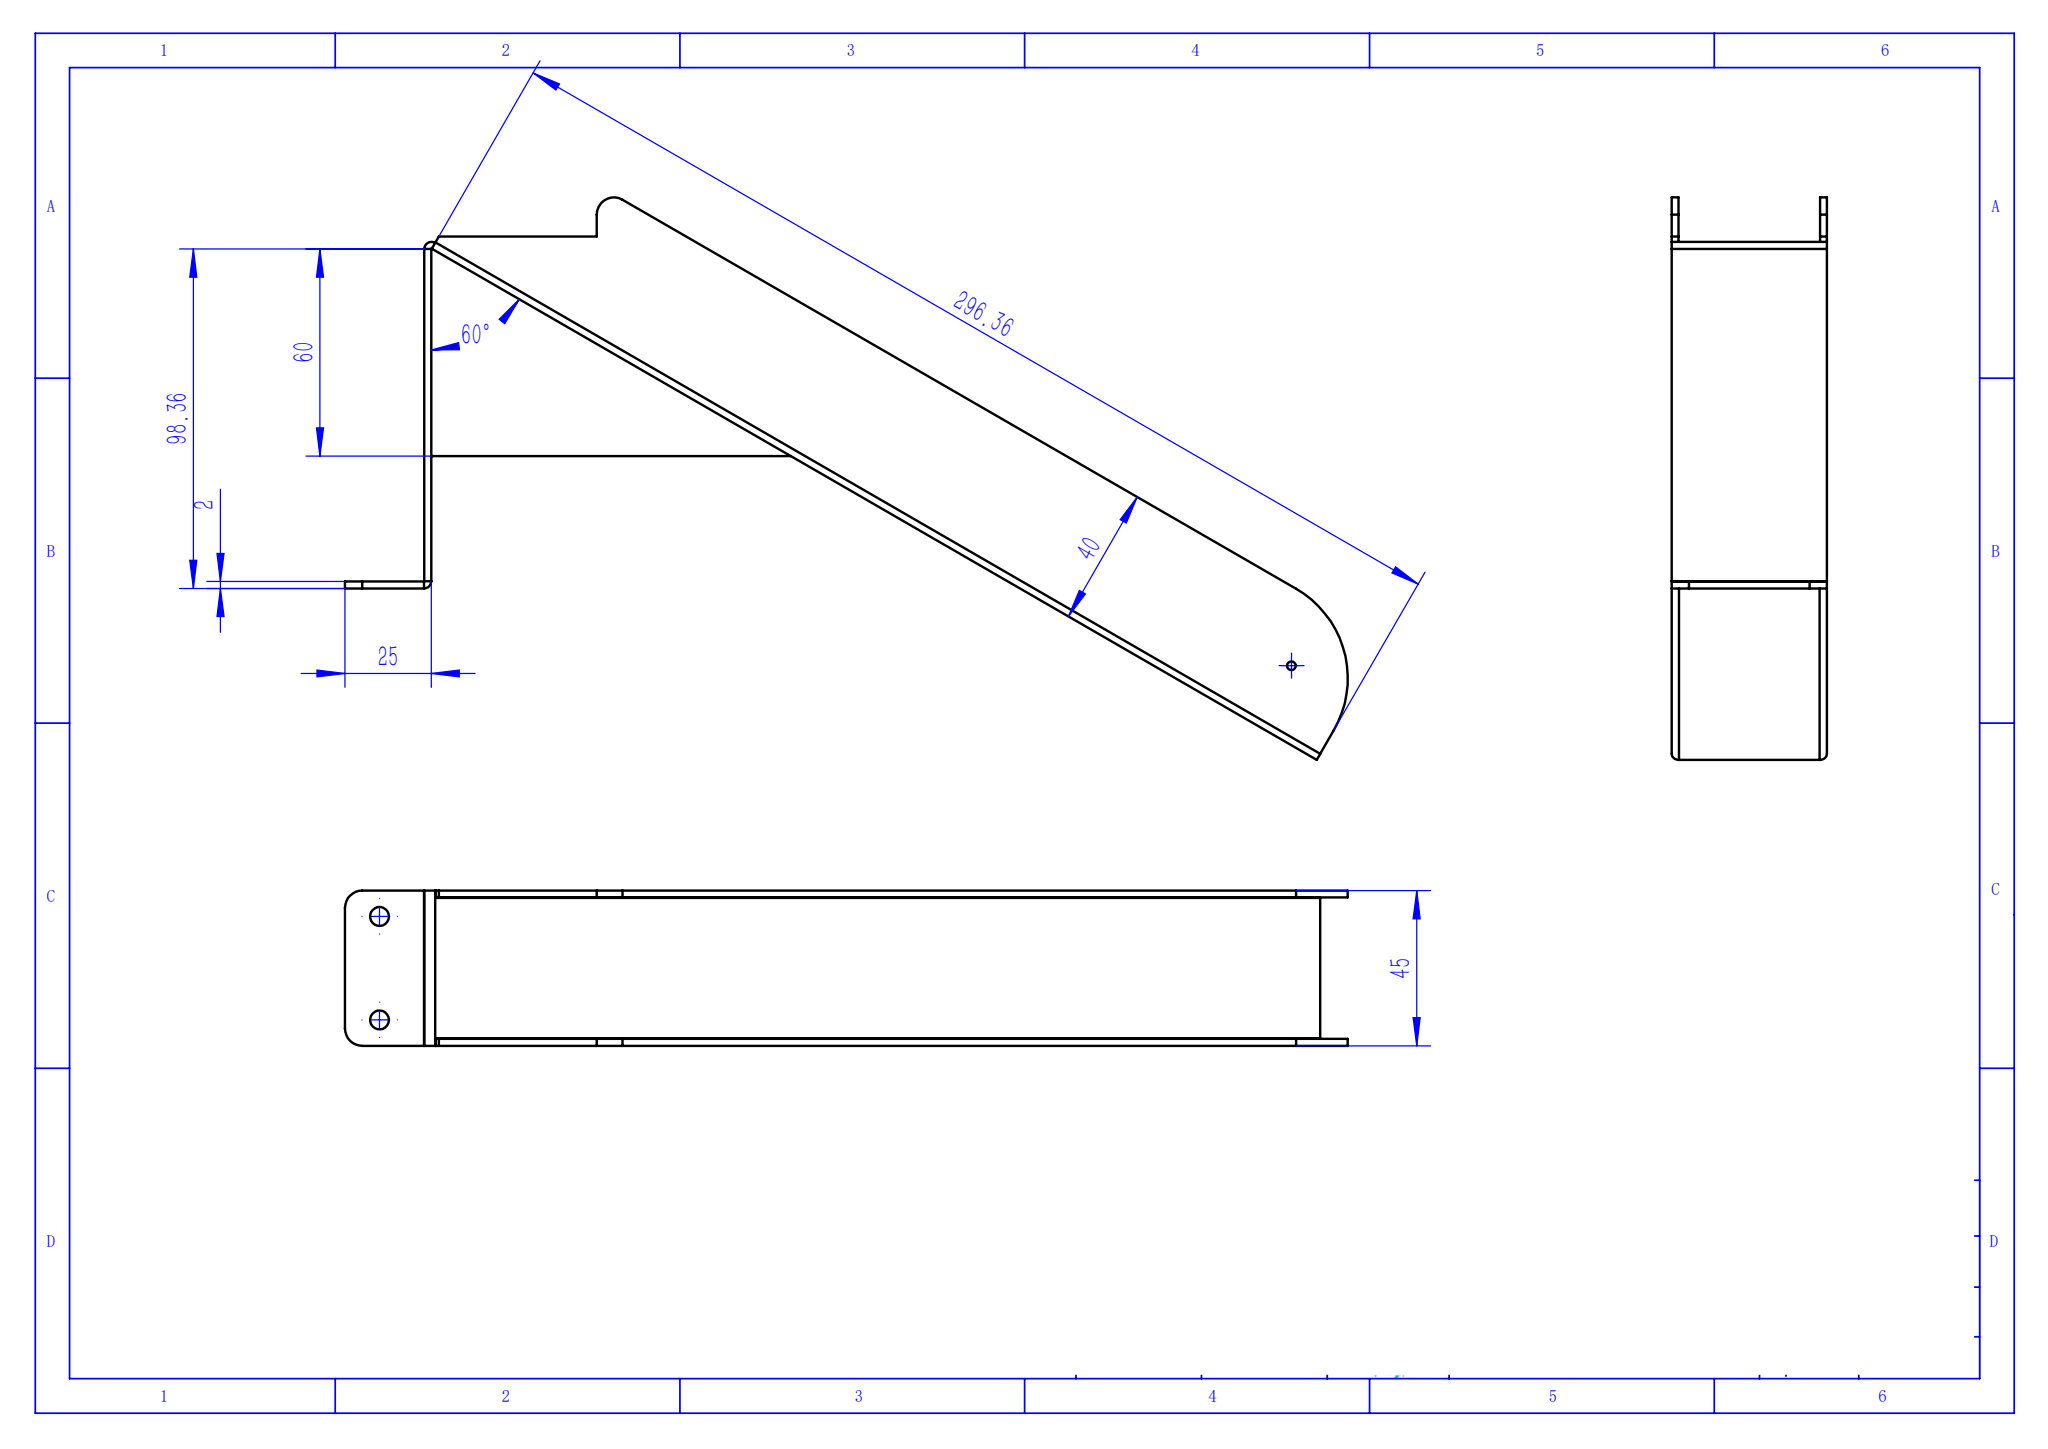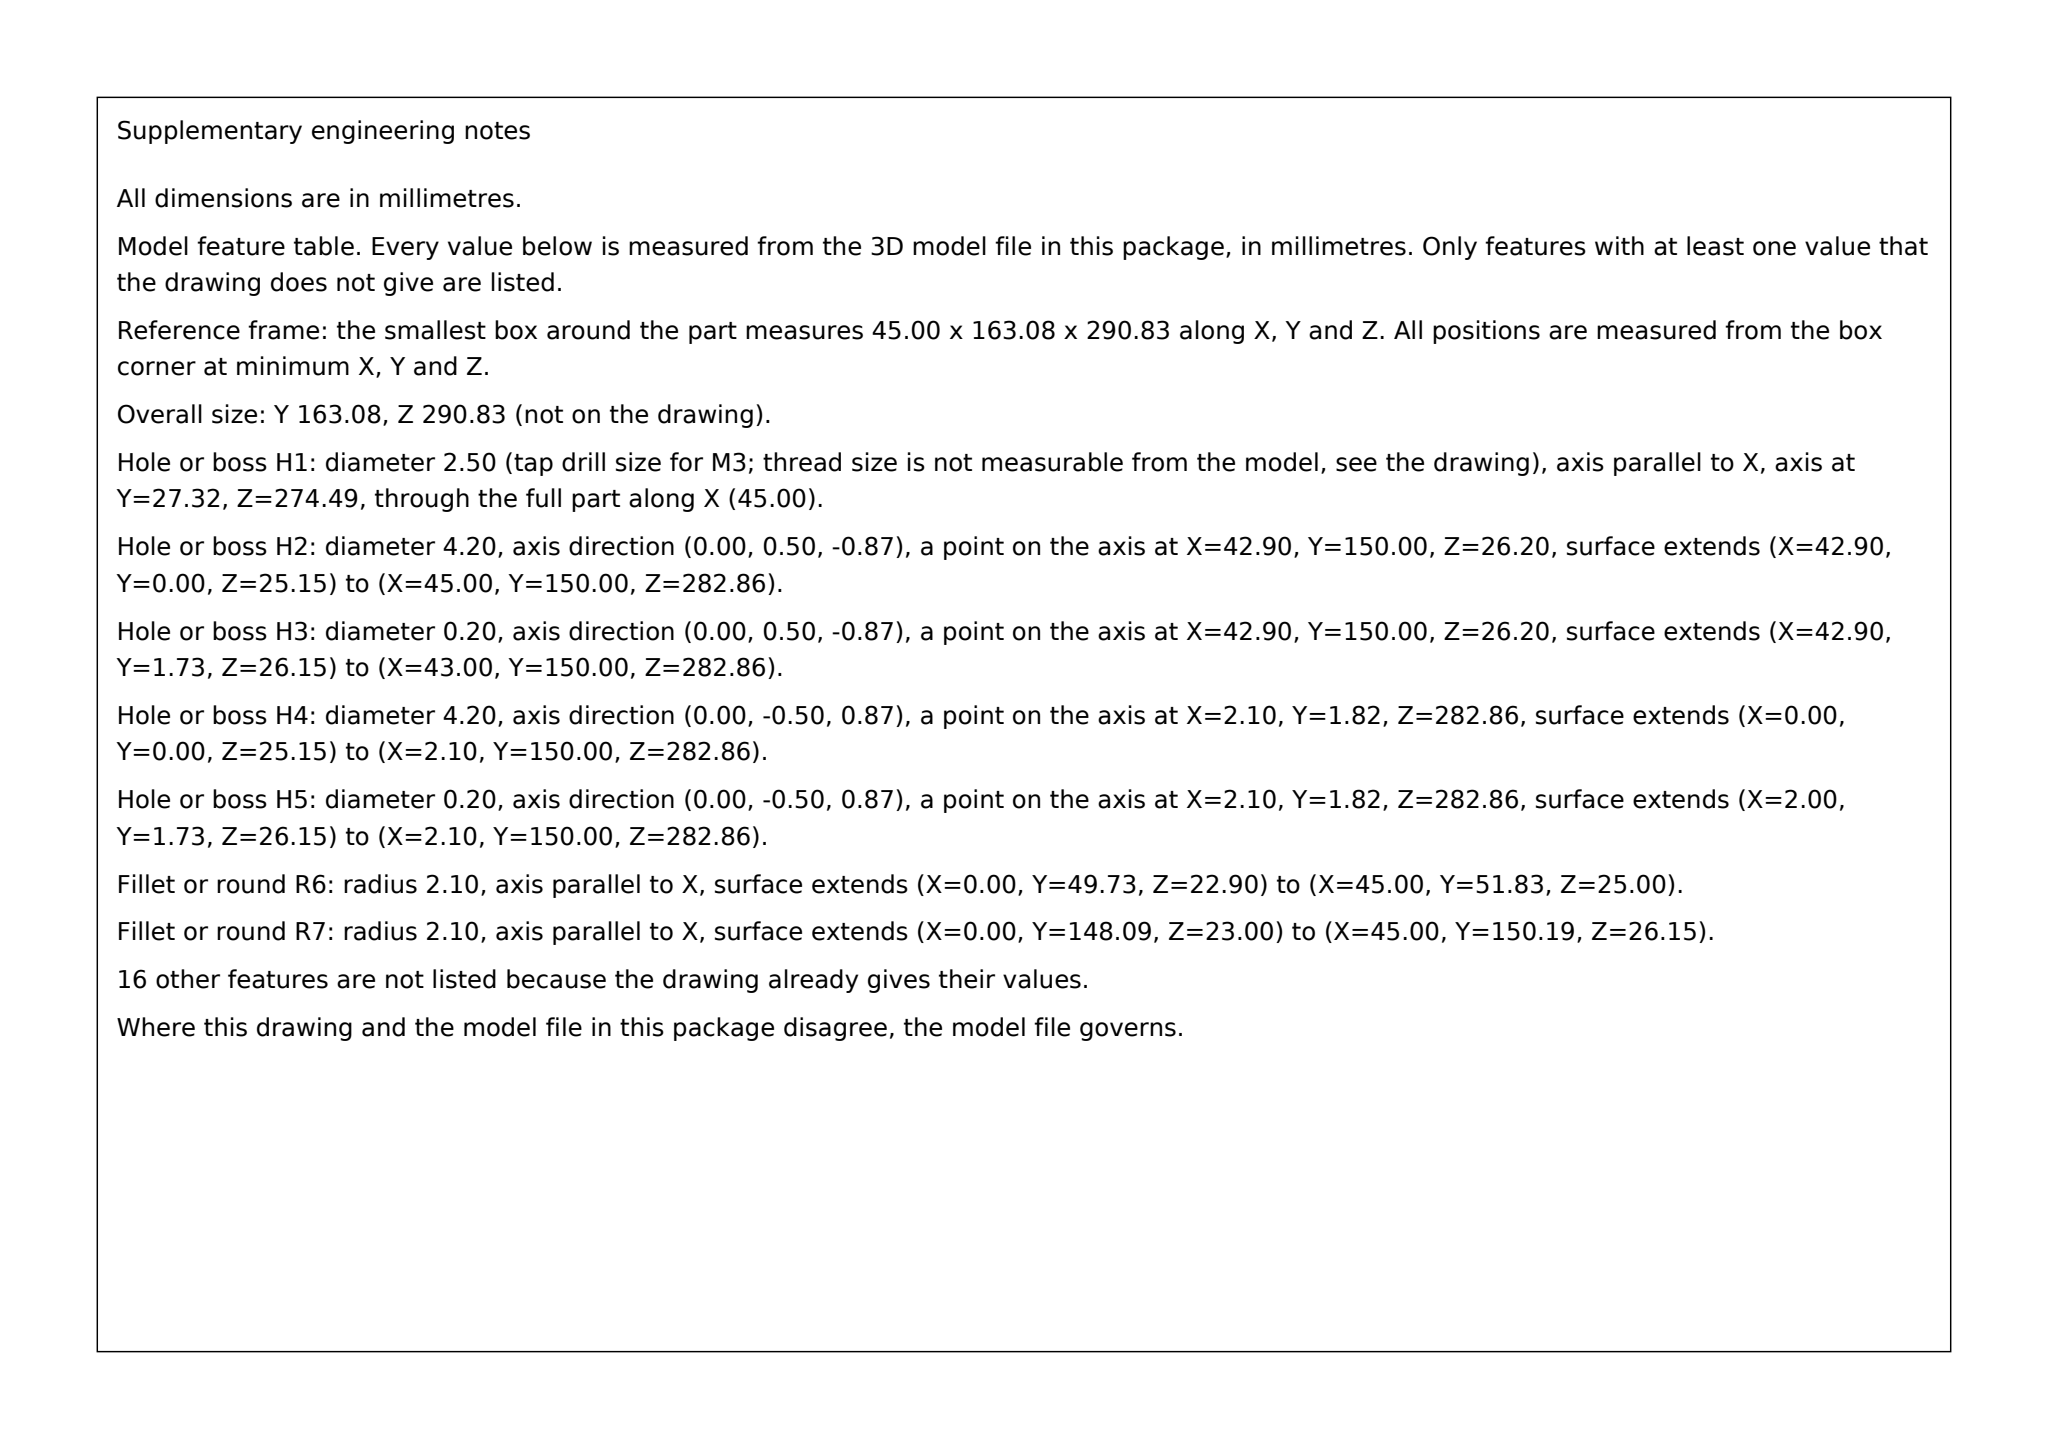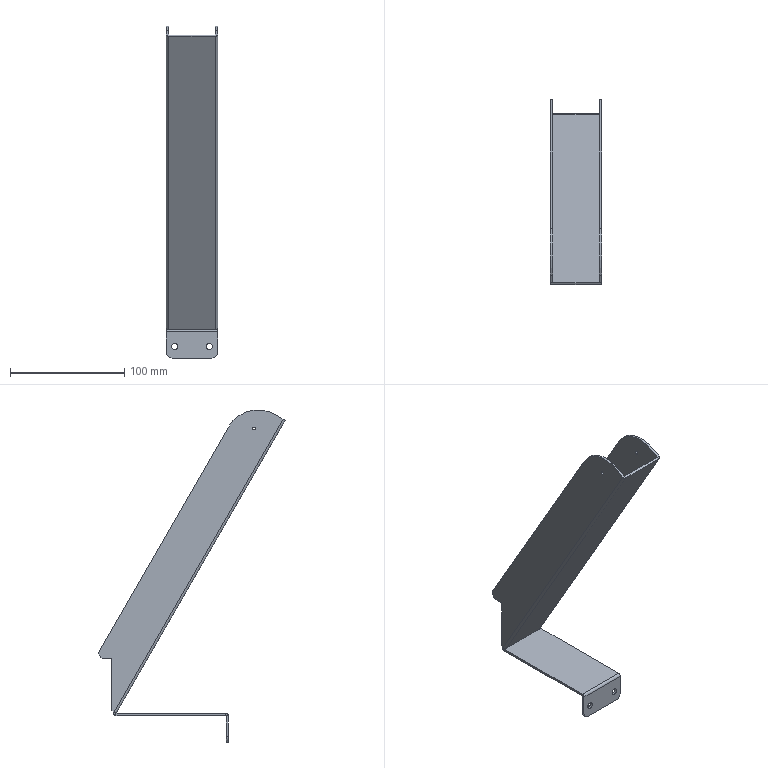Part | SolidWorks | mm | 1 solid | 58 faces | box 45 x 163.08 x 290.83 mm | volume 77586 mm3 | plane 36 | cylinder 22 | commonest cylinder face diameters 2.5 x4 5.5 x4 0.2 x4 4.2 x4 10 x4 60 x2
Drawing notes:
Top flange length 50 mm, measured from the outer face of the vertical leg (z=23) to the flange end before the R5 lip bend (z=73) — value restored from the obscured callout. | from the solid: axis_planes z=23.0 and z=73.0 (flange faces), 10.0 dia x-axis fillet at y=158.08, z=78.0
2X Ø5.5 THRU in the 25 mm bottom flange: hole centres 10 mm from the flange end edge (z=0 datum face), spaced 30 mm apart and symmetric about the 45 mm width (x=7.5 and x=37.5 from the side face). | from the solid: cylinders dia 5.5, y-axis, positions [7.5, -, 10.0] and [37.5, -, 10.0], length 2.0
R30 end radius of the angled brace: centre located 260.83 mm from the back face (z=0) and 23.66 mm from the bottom face (y=0). | from the solid: cylinder dia 60.0, x-axis, pos_other_axes [-, 23.66, 260.83], length 2.0
All dimensions are in millimetres. | from the solid: STEP model facts stated in mm